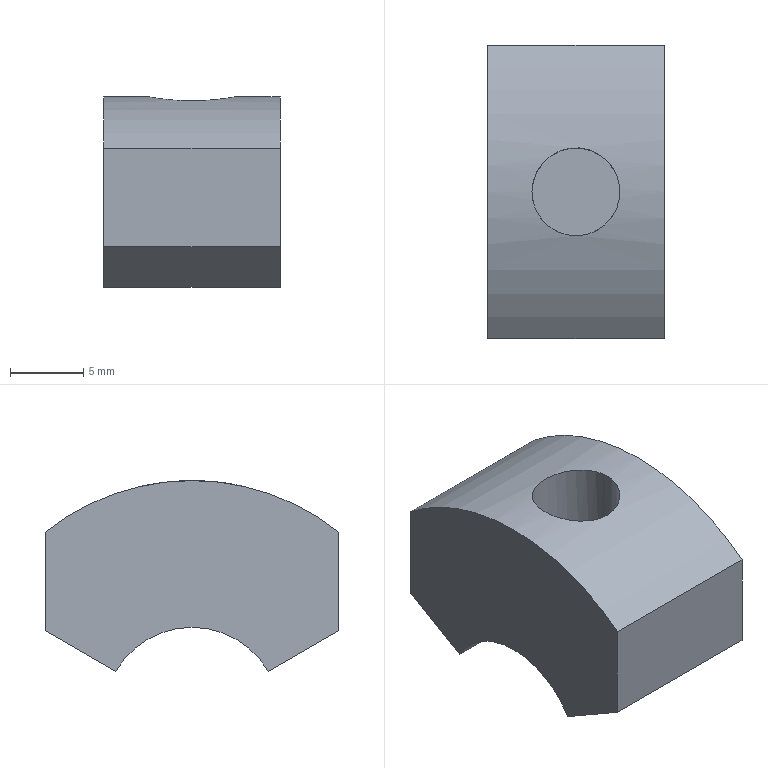Component | NX | BEARING_BUSH | 1 solid | 10 faces | box 12 x 20 x 13 mm | volume 2260 mm3 | plane 7 | cylinder 3 | commonest cylinder face diameters 12 x1 32 x1 6 x1
STEP:
#1=CARTESIAN_POINT('',(0.,0.,0.));
#2=DIRECTION('',(0.,0.,1.));
#3=DIRECTION('',(1.,0.,0.));
#4=AXIS2_PLACEMENT_3D('',#1,#2,#3);
#5=CARTESIAN_POINT('',(6.,10.,48.99));
#6=VERTEX_POINT('',#5);
#7=CARTESIAN_POINT('',(6.,10.,42.274));
#8=VERTEX_POINT('',#7);
#9=CARTESIAN_POINT('',(6.,10.,48.99));
#10=DIRECTION('',(0.,0.,-1.));
#11=VECTOR('',#10,1.);
#12=LINE('',#9,#11);
#13=CARTESIAN_POINT('',(-6.,10.,48.99));
#14=DIRECTION('',(0.,-1.,-0.));
#15=DIRECTION('',(0.,-0.,1.));
#16=AXIS2_PLACEMENT_3D('',#13,#14,#15);
#17=PLANE('',#16);
#18=CARTESIAN_POINT('',(0.,-12.));
#19=DIRECTION('',(-1.,0.));
#20=VECTOR('',#19,1.);
#21=LINE('',#18,#20);
#22=(GEOMETRIC_REPRESENTATION_CONTEXT(2)PARAMETRIC_REPRESENTATION_CONTEXT()REPRESENTATION_CONTEXT('',''));
#23=DEFINITIONAL_REPRESENTATION('',(#21),#22);
#24=PCURVE('',#17,#23);
#25=CARTESIAN_POINT('',(6.,-0.,36.5));
#26=DIRECTION('',(1.,0.,0.));
#27=DIRECTION('',(0.,0.,1.));
#28=AXIS2_PLACEMENT_3D('',#25,#26,#27);
#29=PLANE('',#28);
#30=CARTESIAN_POINT('',(12.49,-10.));
#31=DIRECTION('',(-1.,-0.));
#32=VECTOR('',#31,1.);
#33=LINE('',#30,#32);
#34=(GEOMETRIC_REPRESENTATION_CONTEXT(2)PARAMETRIC_REPRESENTATION_CONTEXT()REPRESENTATION_CONTEXT('',''));
#35=DEFINITIONAL_REPRESENTATION('',(#33),#34);
#36=PCURVE('',#29,#35);
#37=SURFACE_CURVE('',#12,(#24,#36),.PCURVE_S1.);
#38=EDGE_CURVE('',#6,#8,#37,.T.);
#39=ORIENTED_EDGE('',*,*,#38,.T.);
#40=CARTESIAN_POINT('',(-6.,10.,42.274));
#41=VERTEX_POINT('',#40);
#42=CARTESIAN_POINT('',(-6.,10.,42.274));
#43=DIRECTION('',(1.,0.,0.));
#44=VECTOR('',#43,1.);
#45=LINE('',#42,#44);
#46=CARTESIAN_POINT('',(-6.716,0.));
#47=DIRECTION('',(0.,-1.));
#48=VECTOR('',#47,1.);
#49=LINE('',#46,#48);
#50=(GEOMETRIC_REPRESENTATION_CONTEXT(2)PARAMETRIC_REPRESENTATION_CONTEXT()REPRESENTATION_CONTEXT('',''));
#51=DEFINITIONAL_REPRESENTATION('',(#49),#50);
#52=PCURVE('',#17,#51);
#53=CARTESIAN_POINT('',(-6.,10.,42.274));
#54=DIRECTION('',(0.,-0.5,0.866));
#55=DIRECTION('',(0.,0.866,0.5));
#56=AXIS2_PLACEMENT_3D('',#53,#54,#55);
#57=PLANE('',#56);
#58=CARTESIAN_POINT('',(0.,0.));
#59=DIRECTION('',(0.,-1.));
#60=VECTOR('',#59,1.);
#61=LINE('',#58,#60);
#62=(GEOMETRIC_REPRESENTATION_CONTEXT(2)PARAMETRIC_REPRESENTATION_CONTEXT()REPRESENTATION_CONTEXT('',''));
#63=DEFINITIONAL_REPRESENTATION('',(#61),#62);
#64=PCURVE('',#57,#63);
#65=SURFACE_CURVE('',#45,(#52,#64),.PCURVE_S1.);
#66=EDGE_CURVE('',#41,#8,#65,.T.);
#67=ORIENTED_EDGE('',*,*,#66,.F.);
#68=CARTESIAN_POINT('',(-6.,10.,48.99));
#69=VERTEX_POINT('',#68);
#70=CARTESIAN_POINT('',(-6.,10.,48.99));
#71=DIRECTION('',(0.,0.,-1.));
#72=VECTOR('',#71,1.);
#73=LINE('',#70,#72);
#74=CARTESIAN_POINT('',(0.,0.));
#75=DIRECTION('',(-1.,0.));
#76=VECTOR('',#75,1.);
#77=LINE('',#74,#76);
#78=(GEOMETRIC_REPRESENTATION_CONTEXT(2)PARAMETRIC_REPRESENTATION_CONTEXT()REPRESENTATION_CONTEXT('',''));
#79=DEFINITIONAL_REPRESENTATION('',(#77),#78);
#80=PCURVE('',#17,#79);
#81=CARTESIAN_POINT('',(-6.,-0.,36.5));
#82=DIRECTION('',(1.,0.,0.));
#83=DIRECTION('',(0.,0.,1.));
#84=AXIS2_PLACEMENT_3D('',#81,#82,#83);
#85=PLANE('',#84);
#86=CARTESIAN_POINT('',(12.49,-10.));
#87=DIRECTION('',(-1.,-0.));
#88=VECTOR('',#87,1.);
#89=LINE('',#86,#88);
#90=(GEOMETRIC_REPRESENTATION_CONTEXT(2)PARAMETRIC_REPRESENTATION_CONTEXT()REPRESENTATION_CONTEXT('',''));
#91=DEFINITIONAL_REPRESENTATION('',(#89),#90);
#92=PCURVE('',#85,#91);
#93=SURFACE_CURVE('',#73,(#80,#92),.PCURVE_S1.);
#94=EDGE_CURVE('',#69,#41,#93,.T.);
#95=ORIENTED_EDGE('',*,*,#94,.F.);
#96=CARTESIAN_POINT('',(-6.,10.,48.99));
#97=DIRECTION('',(1.,0.,0.));
#98=VECTOR('',#97,1.);
#99=LINE('',#96,#98);
#100=CARTESIAN_POINT('',(0.,0.));
#101=DIRECTION('',(0.,-1.));
#102=VECTOR('',#101,1.);
#103=LINE('',#100,#102);
#104=(GEOMETRIC_REPRESENTATION_CONTEXT(2)PARAMETRIC_REPRESENTATION_CONTEXT()REPRESENTATION_CONTEXT('',''));
#105=DEFINITIONAL_REPRESENTATION('',(#103),#104);
#106=PCURVE('',#17,#105);
#107=CARTESIAN_POINT('',(-6.,-0.,36.5));
#108=DIRECTION('',(1.,0.,0.));
#109=DIRECTION('',(0.,0.,1.));
#110=AXIS2_PLACEMENT_3D('',#107,#108,#109);
#111=CYLINDRICAL_SURFACE('',#110,16.);
#112=CARTESIAN_POINT('',(-0.6751,0.));
#113=DIRECTION('',(0.,1.));
#114=VECTOR('',#113,1.);
#115=LINE('',#112,#114);
#116=(GEOMETRIC_REPRESENTATION_CONTEXT(2)PARAMETRIC_REPRESENTATION_CONTEXT()REPRESENTATION_CONTEXT('',''));
#117=DEFINITIONAL_REPRESENTATION('',(#115),#116);
#118=PCURVE('',#111,#117);
#119=SURFACE_CURVE('',#99,(#106,#118),.PCURVE_S1.);
#120=EDGE_CURVE('',#69,#6,#119,.T.);
#121=ORIENTED_EDGE('',*,*,#120,.T.);
#122=EDGE_LOOP('',(#39,#67,#95,#121));
#123=FACE_BOUND('',#122,.T.);
#124=ADVANCED_FACE('',(#123),#17,.F.);
#125=CARTESIAN_POINT('',(6.,5.196,39.5));
#126=VERTEX_POINT('',#125);
#127=CARTESIAN_POINT('',(6.,10.,42.274));
#128=DIRECTION('',(0.,-0.866,-0.5));
#129=VECTOR('',#128,1.);
#130=LINE('',#127,#129);
#131=CARTESIAN_POINT('',(0.,-12.));
#132=DIRECTION('',(-1.,0.));
#133=VECTOR('',#132,1.);
#134=LINE('',#131,#133);
#135=(GEOMETRIC_REPRESENTATION_CONTEXT(2)PARAMETRIC_REPRESENTATION_CONTEXT()REPRESENTATION_CONTEXT('',''));
#136=DEFINITIONAL_REPRESENTATION('',(#134),#135);
#137=PCURVE('',#57,#136);
#138=CARTESIAN_POINT('',(5.774,-10.));
#139=DIRECTION('',(-0.5,0.866));
#140=VECTOR('',#139,1.);
#141=LINE('',#138,#140);
#142=(GEOMETRIC_REPRESENTATION_CONTEXT(2)PARAMETRIC_REPRESENTATION_CONTEXT()REPRESENTATION_CONTEXT('',''));
#143=DEFINITIONAL_REPRESENTATION('',(#141),#142);
#144=PCURVE('',#29,#143);
#145=SURFACE_CURVE('',#130,(#137,#144),.PCURVE_S1.);
#146=EDGE_CURVE('',#8,#126,#145,.T.);
#147=ORIENTED_EDGE('',*,*,#146,.T.);
#148=CARTESIAN_POINT('',(-6.,5.196,39.5));
#149=VERTEX_POINT('',#148);
#150=CARTESIAN_POINT('',(-6.,5.196,39.5));
#151=DIRECTION('',(1.,0.,0.));
#152=VECTOR('',#151,1.);
#153=LINE('',#150,#152);
#154=CARTESIAN_POINT('',(-5.547,0.));
#155=DIRECTION('',(0.,-1.));
#156=VECTOR('',#155,1.);
#157=LINE('',#154,#156);
#158=(GEOMETRIC_REPRESENTATION_CONTEXT(2)PARAMETRIC_REPRESENTATION_CONTEXT()REPRESENTATION_CONTEXT('',''));
#159=DEFINITIONAL_REPRESENTATION('',(#157),#158);
#160=PCURVE('',#57,#159);
#161=CARTESIAN_POINT('',(-6.,-0.,36.5));
#162=DIRECTION('',(1.,0.,0.));
#163=DIRECTION('',(0.,0.,1.));
#164=AXIS2_PLACEMENT_3D('',#161,#162,#163);
#165=CYLINDRICAL_SURFACE('',#164,6.);
#166=CARTESIAN_POINT('',(5.236,0.));
#167=DIRECTION('',(0.,1.));
#168=VECTOR('',#167,1.);
#169=LINE('',#166,#168);
#170=(GEOMETRIC_REPRESENTATION_CONTEXT(2)PARAMETRIC_REPRESENTATION_CONTEXT()REPRESENTATION_CONTEXT('',''));
#171=DEFINITIONAL_REPRESENTATION('',(#169),#170);
#172=PCURVE('',#165,#171);
#173=SURFACE_CURVE('',#153,(#160,#172),.PCURVE_S1.);
#174=EDGE_CURVE('',#149,#126,#173,.T.);
#175=ORIENTED_EDGE('',*,*,#174,.F.);
#176=CARTESIAN_POINT('',(-6.,10.,42.274));
#177=DIRECTION('',(0.,-0.866,-0.5));
#178=VECTOR('',#177,1.);
#179=LINE('',#176,#178);
#180=CARTESIAN_POINT('',(0.,0.));
#181=DIRECTION('',(-1.,0.));
#182=VECTOR('',#181,1.);
#183=LINE('',#180,#182);
#184=(GEOMETRIC_REPRESENTATION_CONTEXT(2)PARAMETRIC_REPRESENTATION_CONTEXT()REPRESENTATION_CONTEXT('',''));
#185=DEFINITIONAL_REPRESENTATION('',(#183),#184);
#186=PCURVE('',#57,#185);
#187=CARTESIAN_POINT('',(5.774,-10.));
#188=DIRECTION('',(-0.5,0.866));
#189=VECTOR('',#188,1.);
#190=LINE('',#187,#189);
#191=(GEOMETRIC_REPRESENTATION_CONTEXT(2)PARAMETRIC_REPRESENTATION_CONTEXT()REPRESENTATION_CONTEXT('',''));
#192=DEFINITIONAL_REPRESENTATION('',(#190),#191);
#193=PCURVE('',#85,#192);
#194=SURFACE_CURVE('',#179,(#186,#193),.PCURVE_S1.);
#195=EDGE_CURVE('',#41,#149,#194,.T.);
#196=ORIENTED_EDGE('',*,*,#195,.F.);
#197=ORIENTED_EDGE('',*,*,#66,.T.);
#198=EDGE_LOOP('',(#147,#175,#196,#197));
#199=FACE_BOUND('',#198,.T.);
#200=ADVANCED_FACE('',(#199),#57,.F.);
#201=ORIENTED_EDGE('',*,*,#174,.F.);
#202=CARTESIAN_POINT('',(-6.,-5.196,39.5));
#203=VERTEX_POINT('',#202);
#204=CARTESIAN_POINT('',(-6.,-0.,36.5));
#205=DIRECTION('',(1.,0.,0.));
#206=DIRECTION('',(0.,-1.,0.));
#207=AXIS2_PLACEMENT_3D('',#204,#205,#206);
#208=CIRCLE('',#207,6.);
#209=CARTESIAN_POINT('',(1.571,0.));
#210=DIRECTION('',(1.,0.));
#211=VECTOR('',#210,1.);
#212=LINE('',#209,#211);
#213=(GEOMETRIC_REPRESENTATION_CONTEXT(2)PARAMETRIC_REPRESENTATION_CONTEXT()REPRESENTATION_CONTEXT('',''));
#214=DEFINITIONAL_REPRESENTATION('',(#212),#213);
#215=PCURVE('',#165,#214);
#216=CARTESIAN_POINT('',(0.,0.));
#217=DIRECTION('',(0.,1.));
#218=AXIS2_PLACEMENT_2D('',#216,#217);
#219=CIRCLE('',#218,6.);
#220=(GEOMETRIC_REPRESENTATION_CONTEXT(2)PARAMETRIC_REPRESENTATION_CONTEXT()REPRESENTATION_CONTEXT('',''));
#221=DEFINITIONAL_REPRESENTATION('',(#219),#220);
#222=PCURVE('',#85,#221);
#223=SURFACE_CURVE('',#208,(#215,#222),.PCURVE_S1.);
#224=EDGE_CURVE('',#149,#203,#223,.T.);
#225=ORIENTED_EDGE('',*,*,#224,.T.);
#226=CARTESIAN_POINT('',(6.,-5.196,39.5));
#227=VERTEX_POINT('',#226);
#228=CARTESIAN_POINT('',(-6.,-5.196,39.5));
#229=DIRECTION('',(1.,0.,0.));
#230=VECTOR('',#229,1.);
#231=LINE('',#228,#230);
#232=CARTESIAN_POINT('',(7.33,0.));
#233=DIRECTION('',(0.,1.));
#234=VECTOR('',#233,1.);
#235=LINE('',#232,#234);
#236=(GEOMETRIC_REPRESENTATION_CONTEXT(2)PARAMETRIC_REPRESENTATION_CONTEXT()REPRESENTATION_CONTEXT('',''));
#237=DEFINITIONAL_REPRESENTATION('',(#235),#236);
#238=PCURVE('',#165,#237);
#239=CARTESIAN_POINT('',(-6.,-5.196,39.5));
#240=DIRECTION('',(0.,0.5,0.866));
#241=DIRECTION('',(0.,0.866,-0.5));
#242=AXIS2_PLACEMENT_3D('',#239,#240,#241);
#243=PLANE('',#242);
#244=CARTESIAN_POINT('',(0.,0.));
#245=DIRECTION('',(0.,-1.));
#246=VECTOR('',#245,1.);
#247=LINE('',#244,#246);
#248=(GEOMETRIC_REPRESENTATION_CONTEXT(2)PARAMETRIC_REPRESENTATION_CONTEXT()REPRESENTATION_CONTEXT('',''));
#249=DEFINITIONAL_REPRESENTATION('',(#247),#248);
#250=PCURVE('',#243,#249);
#251=SURFACE_CURVE('',#231,(#238,#250),.PCURVE_S1.);
#252=EDGE_CURVE('',#203,#227,#251,.T.);
#253=ORIENTED_EDGE('',*,*,#252,.T.);
#254=CARTESIAN_POINT('',(6.,-0.,36.5));
#255=DIRECTION('',(1.,0.,0.));
#256=DIRECTION('',(0.,-1.,0.));
#257=AXIS2_PLACEMENT_3D('',#254,#255,#256);
#258=CIRCLE('',#257,6.);
#259=CARTESIAN_POINT('',(1.571,12.));
#260=DIRECTION('',(1.,0.));
#261=VECTOR('',#260,1.);
#262=LINE('',#259,#261);
#263=(GEOMETRIC_REPRESENTATION_CONTEXT(2)PARAMETRIC_REPRESENTATION_CONTEXT()REPRESENTATION_CONTEXT('',''));
#264=DEFINITIONAL_REPRESENTATION('',(#262),#263);
#265=PCURVE('',#165,#264);
#266=CARTESIAN_POINT('',(0.,0.));
#267=DIRECTION('',(0.,1.));
#268=AXIS2_PLACEMENT_2D('',#266,#267);
#269=CIRCLE('',#268,6.);
#270=(GEOMETRIC_REPRESENTATION_CONTEXT(2)PARAMETRIC_REPRESENTATION_CONTEXT()REPRESENTATION_CONTEXT('',''));
#271=DEFINITIONAL_REPRESENTATION('',(#269),#270);
#272=PCURVE('',#29,#271);
#273=SURFACE_CURVE('',#258,(#265,#272),.PCURVE_S1.);
#274=EDGE_CURVE('',#126,#227,#273,.T.);
#275=ORIENTED_EDGE('',*,*,#274,.F.);
#276=EDGE_LOOP('',(#201,#225,#253,#275));
#277=FACE_BOUND('',#276,.F.);
#278=ADVANCED_FACE('',(#277),#165,.F.);
#279=CARTESIAN_POINT('',(6.,-10.,42.274));
#280=VERTEX_POINT('',#279);
#281=CARTESIAN_POINT('',(6.,-5.196,39.5));
#282=DIRECTION('',(0.,-0.866,0.5));
#283=VECTOR('',#282,1.);
#284=LINE('',#281,#283);
#285=CARTESIAN_POINT('',(0.,-12.));
#286=DIRECTION('',(-1.,0.));
#287=VECTOR('',#286,1.);
#288=LINE('',#285,#287);
#289=(GEOMETRIC_REPRESENTATION_CONTEXT(2)PARAMETRIC_REPRESENTATION_CONTEXT()REPRESENTATION_CONTEXT('',''));
#290=DEFINITIONAL_REPRESENTATION('',(#288),#289);
#291=PCURVE('',#243,#290);
#292=CARTESIAN_POINT('',(3.,5.196));
#293=DIRECTION('',(0.5,0.866));
#294=VECTOR('',#293,1.);
#295=LINE('',#292,#294);
#296=(GEOMETRIC_REPRESENTATION_CONTEXT(2)PARAMETRIC_REPRESENTATION_CONTEXT()REPRESENTATION_CONTEXT('',''));
#297=DEFINITIONAL_REPRESENTATION('',(#295),#296);
#298=PCURVE('',#29,#297);
#299=SURFACE_CURVE('',#284,(#291,#298),.PCURVE_S1.);
#300=EDGE_CURVE('',#227,#280,#299,.T.);
#301=ORIENTED_EDGE('',*,*,#300,.T.);
#302=CARTESIAN_POINT('',(-6.,-10.,42.274));
#303=VERTEX_POINT('',#302);
#304=CARTESIAN_POINT('',(-6.,-10.,42.274));
#305=DIRECTION('',(1.,0.,0.));
#306=VECTOR('',#305,1.);
#307=LINE('',#304,#306);
#308=CARTESIAN_POINT('',(-5.547,0.));
#309=DIRECTION('',(0.,-1.));
#310=VECTOR('',#309,1.);
#311=LINE('',#308,#310);
#312=(GEOMETRIC_REPRESENTATION_CONTEXT(2)PARAMETRIC_REPRESENTATION_CONTEXT()REPRESENTATION_CONTEXT('',''));
#313=DEFINITIONAL_REPRESENTATION('',(#311),#312);
#314=PCURVE('',#243,#313);
#315=CARTESIAN_POINT('',(-6.,-10.,42.274));
#316=DIRECTION('',(0.,1.,-0.));
#317=DIRECTION('',(0.,-0.,-1.));
#318=AXIS2_PLACEMENT_3D('',#315,#316,#317);
#319=PLANE('',#318);
#320=CARTESIAN_POINT('',(0.,0.));
#321=DIRECTION('',(0.,-1.));
#322=VECTOR('',#321,1.);
#323=LINE('',#320,#322);
#324=(GEOMETRIC_REPRESENTATION_CONTEXT(2)PARAMETRIC_REPRESENTATION_CONTEXT()REPRESENTATION_CONTEXT('',''));
#325=DEFINITIONAL_REPRESENTATION('',(#323),#324);
#326=PCURVE('',#319,#325);
#327=SURFACE_CURVE('',#307,(#314,#326),.PCURVE_S1.);
#328=EDGE_CURVE('',#303,#280,#327,.T.);
#329=ORIENTED_EDGE('',*,*,#328,.F.);
#330=CARTESIAN_POINT('',(-6.,-5.196,39.5));
#331=DIRECTION('',(0.,-0.866,0.5));
#332=VECTOR('',#331,1.);
#333=LINE('',#330,#332);
#334=CARTESIAN_POINT('',(0.,0.));
#335=DIRECTION('',(-1.,0.));
#336=VECTOR('',#335,1.);
#337=LINE('',#334,#336);
#338=(GEOMETRIC_REPRESENTATION_CONTEXT(2)PARAMETRIC_REPRESENTATION_CONTEXT()REPRESENTATION_CONTEXT('',''));
#339=DEFINITIONAL_REPRESENTATION('',(#337),#338);
#340=PCURVE('',#243,#339);
#341=CARTESIAN_POINT('',(3.,5.196));
#342=DIRECTION('',(0.5,0.866));
#343=VECTOR('',#342,1.);
#344=LINE('',#341,#343);
#345=(GEOMETRIC_REPRESENTATION_CONTEXT(2)PARAMETRIC_REPRESENTATION_CONTEXT()REPRESENTATION_CONTEXT('',''));
#346=DEFINITIONAL_REPRESENTATION('',(#344),#345);
#347=PCURVE('',#85,#346);
#348=SURFACE_CURVE('',#333,(#340,#347),.PCURVE_S1.);
#349=EDGE_CURVE('',#203,#303,#348,.T.);
#350=ORIENTED_EDGE('',*,*,#349,.F.);
#351=ORIENTED_EDGE('',*,*,#252,.T.);
#352=EDGE_LOOP('',(#301,#329,#350,#351));
#353=FACE_BOUND('',#352,.T.);
#354=ADVANCED_FACE('',(#353),#243,.F.);
#355=CARTESIAN_POINT('',(6.,-10.,48.99));
#356=VERTEX_POINT('',#355);
#357=CARTESIAN_POINT('',(6.,-10.,42.274));
#358=DIRECTION('',(0.,0.,1.));
#359=VECTOR('',#358,1.);
#360=LINE('',#357,#359);
#361=CARTESIAN_POINT('',(0.,-12.));
#362=DIRECTION('',(-1.,0.));
#363=VECTOR('',#362,1.);
#364=LINE('',#361,#363);
#365=(GEOMETRIC_REPRESENTATION_CONTEXT(2)PARAMETRIC_REPRESENTATION_CONTEXT()REPRESENTATION_CONTEXT('',''));
#366=DEFINITIONAL_REPRESENTATION('',(#364),#365);
#367=PCURVE('',#319,#366);
#368=CARTESIAN_POINT('',(5.774,10.));
#369=DIRECTION('',(1.,-0.));
#370=VECTOR('',#369,1.);
#371=LINE('',#368,#370);
#372=(GEOMETRIC_REPRESENTATION_CONTEXT(2)PARAMETRIC_REPRESENTATION_CONTEXT()REPRESENTATION_CONTEXT('',''));
#373=DEFINITIONAL_REPRESENTATION('',(#371),#372);
#374=PCURVE('',#29,#373);
#375=SURFACE_CURVE('',#360,(#367,#374),.PCURVE_S1.);
#376=EDGE_CURVE('',#280,#356,#375,.T.);
#377=ORIENTED_EDGE('',*,*,#376,.T.);
#378=CARTESIAN_POINT('',(-6.,-10.,48.99));
#379=VERTEX_POINT('',#378);
#380=CARTESIAN_POINT('',(-6.,-10.,48.99));
#381=DIRECTION('',(1.,0.,0.));
#382=VECTOR('',#381,1.);
#383=LINE('',#380,#382);
#384=CARTESIAN_POINT('',(-6.716,0.));
#385=DIRECTION('',(0.,-1.));
#386=VECTOR('',#385,1.);
#387=LINE('',#384,#386);
#388=(GEOMETRIC_REPRESENTATION_CONTEXT(2)PARAMETRIC_REPRESENTATION_CONTEXT()REPRESENTATION_CONTEXT('',''));
#389=DEFINITIONAL_REPRESENTATION('',(#387),#388);
#390=PCURVE('',#319,#389);
#391=CARTESIAN_POINT('',(0.6751,0.));
#392=DIRECTION('',(0.,1.));
#393=VECTOR('',#392,1.);
#394=LINE('',#391,#393);
#395=(GEOMETRIC_REPRESENTATION_CONTEXT(2)PARAMETRIC_REPRESENTATION_CONTEXT()REPRESENTATION_CONTEXT('',''));
#396=DEFINITIONAL_REPRESENTATION('',(#394),#395);
#397=PCURVE('',#111,#396);
#398=SURFACE_CURVE('',#383,(#390,#397),.PCURVE_S1.);
#399=EDGE_CURVE('',#379,#356,#398,.T.);
#400=ORIENTED_EDGE('',*,*,#399,.F.);
#401=CARTESIAN_POINT('',(-6.,-10.,42.274));
#402=DIRECTION('',(0.,0.,1.));
#403=VECTOR('',#402,1.);
#404=LINE('',#401,#403);
#405=CARTESIAN_POINT('',(0.,0.));
#406=DIRECTION('',(-1.,0.));
#407=VECTOR('',#406,1.);
#408=LINE('',#405,#407);
#409=(GEOMETRIC_REPRESENTATION_CONTEXT(2)PARAMETRIC_REPRESENTATION_CONTEXT()REPRESENTATION_CONTEXT('',''));
#410=DEFINITIONAL_REPRESENTATION('',(#408),#409);
#411=PCURVE('',#319,#410);
#412=CARTESIAN_POINT('',(5.774,10.));
#413=DIRECTION('',(1.,-0.));
#414=VECTOR('',#413,1.);
#415=LINE('',#412,#414);
#416=(GEOMETRIC_REPRESENTATION_CONTEXT(2)PARAMETRIC_REPRESENTATION_CONTEXT()REPRESENTATION_CONTEXT('',''));
#417=DEFINITIONAL_REPRESENTATION('',(#415),#416);
#418=PCURVE('',#85,#417);
#419=SURFACE_CURVE('',#404,(#411,#418),.PCURVE_S1.);
#420=EDGE_CURVE('',#303,#379,#419,.T.);
#421=ORIENTED_EDGE('',*,*,#420,.F.);
#422=ORIENTED_EDGE('',*,*,#328,.T.);
#423=EDGE_LOOP('',(#377,#400,#421,#422));
#424=FACE_BOUND('',#423,.T.);
#425=ADVANCED_FACE('',(#424),#319,.F.);
#426=CARTESIAN_POINT('',(-3.,-0.,52.5));
#427=VERTEX_POINT('',#426);
#428=CARTESIAN_POINT('',(-3.,-0.,52.5));
#429=CARTESIAN_POINT('',(-3.,0.3325,52.5));
#430=CARTESIAN_POINT('',(-2.943,0.6696,52.489));
#431=CARTESIAN_POINT('',(-2.834,0.9833,52.47));
#432=CARTESIAN_POINT('',(-2.726,1.297,52.45));
#433=CARTESIAN_POINT('',(-2.562,1.595,52.422));
#434=CARTESIAN_POINT('',(-2.357,1.856,52.392));
#435=CARTESIAN_POINT('',(-2.15,2.118,52.361));
#436=CARTESIAN_POINT('',(-1.896,2.349,52.328));
#437=CARTESIAN_POINT('',(-1.614,2.529,52.299));
#438=CARTESIAN_POINT('',(-1.329,2.711,52.27));
#439=CARTESIAN_POINT('',(-1.009,2.845,52.245));
#440=CARTESIAN_POINT('',(-0.6794,2.922,52.231));
#441=CARTESIAN_POINT('',(-0.3538,2.998,52.217));
#442=CARTESIAN_POINT('',(-0.01006,3.019,52.213));
#443=CARTESIAN_POINT('',(0.3225,2.983,52.22));
#444=CARTESIAN_POINT('',(0.6508,2.947,52.226));
#445=CARTESIAN_POINT('',(0.9772,2.855,52.244));
#446=CARTESIAN_POINT('',(1.275,2.715,52.268));
#447=CARTESIAN_POINT('',(1.575,2.575,52.292));
#448=CARTESIAN_POINT('',(1.855,2.381,52.324));
#449=CARTESIAN_POINT('',(2.092,2.15,52.355));
#450=CARTESIAN_POINT('',(2.333,1.916,52.387));
#451=CARTESIAN_POINT('',(2.536,1.637,52.419));
#452=CARTESIAN_POINT('',(2.686,1.336,52.444));
#453=CARTESIAN_POINT('',(2.836,1.034,52.469));
#454=CARTESIAN_POINT('',(2.936,0.7015,52.488));
#455=CARTESIAN_POINT('',(2.978,0.3662,52.496));
#456=CARTESIAN_POINT('',(3.018,0.03596,52.503));
#457=CARTESIAN_POINT('',(3.003,-0.3061,52.5));
#458=CARTESIAN_POINT('',(2.933,-0.6313,52.488));
#459=CARTESIAN_POINT('',(2.863,-0.9539,52.475));
#460=CARTESIAN_POINT('',(2.738,-1.269,52.452));
#461=CARTESIAN_POINT('',(2.568,-1.551,52.425));
#462=CARTESIAN_POINT('',(2.396,-1.835,52.397));
#463=CARTESIAN_POINT('',(2.173,-2.094,52.364));
#464=CARTESIAN_POINT('',(1.918,-2.307,52.333));
#465=CARTESIAN_POINT('',(1.659,-2.522,52.301));
#466=CARTESIAN_POINT('',(1.359,-2.696,52.272));
#467=CARTESIAN_POINT('',(1.042,-2.813,52.251));
#468=CARTESIAN_POINT('',(0.7268,-2.93,52.23));
#469=CARTESIAN_POINT('',(0.3865,-2.994,52.217));
#470=CARTESIAN_POINT('',(0.04993,-3.,52.216));
#471=CARTESIAN_POINT('',(-0.2813,-3.005,52.215));
#472=CARTESIAN_POINT('',(-0.6181,-2.954,52.225));
#473=CARTESIAN_POINT('',(-0.9325,-2.851,52.244));
#474=CARTESIAN_POINT('',(-1.246,-2.749,52.262));
#475=CARTESIAN_POINT('',(-1.546,-2.592,52.29));
#476=CARTESIAN_POINT('',(-1.809,-2.393,52.32));
#477=CARTESIAN_POINT('',(-2.076,-2.191,52.351));
#478=CARTESIAN_POINT('',(-2.311,-1.941,52.384));
#479=CARTESIAN_POINT('',(-2.497,-1.663,52.413));
#480=CARTESIAN_POINT('',(-2.684,-1.382,52.443));
#481=CARTESIAN_POINT('',(-2.825,-1.065,52.468));
#482=CARTESIAN_POINT('',(-2.908,-0.7369,52.483));
#483=CARTESIAN_POINT('',(-2.969,-0.4971,52.494));
#484=CARTESIAN_POINT('',(-3.,-0.2476,52.5));
#485=CARTESIAN_POINT('',(-3.,-0.,52.5));
#486=B_SPLINE_CURVE_WITH_KNOTS('',3,(#428,#429,#430,#431,#432,#433,#434,#435,#436,#437,#438,#439,#440,#441,#442,#443,#444,#445,#446,#447,#448,#449,#450,#451,#452,#453,#454,#455,#456,#457,#458,#459,#460,#461,#462,#463,#464,#465,#466,#467,#468,#469,#470,#471,#472,#473,#474,#475,#476,#477,#478,#479,#480,#481,#482,#483,#484,#485),.UNSPECIFIED.,.T.,.F.,(1,3,3,3,3,3,3,3,3,3,3,3,3,3,3,3,3,3,3,3,3,1),(-0.03926,0.,0.05307,0.1061,0.1597,0.2138,0.2672,0.3199,0.3729,0.4267,0.4807,0.5338,0.5865,0.6397,0.6938,0.7475,0.8004,0.8531,0.9067,0.9607,1.,1.053),.UNSPECIFIED.);
#487=CARTESIAN_POINT('',(0.,3.));
#488=CARTESIAN_POINT('',(-0.00445,3.));
#489=CARTESIAN_POINT('',(-0.01338,3.005));
#490=CARTESIAN_POINT('',(-0.02675,3.028));
#491=CARTESIAN_POINT('',(-0.03999,3.067));
#492=CARTESIAN_POINT('',(-0.05301,3.12));
#493=CARTESIAN_POINT('',(-0.06569,3.187));
#494=CARTESIAN_POINT('',(-0.07809,3.269));
#495=CARTESIAN_POINT('',(-0.09012,3.366));
#496=CARTESIAN_POINT('',(-0.1017,3.475));
#497=CARTESIAN_POINT('',(-0.1128,3.597));
#498=CARTESIAN_POINT('',(-0.1232,3.731));
#499=CARTESIAN_POINT('',(-0.133,3.877));
#500=CARTESIAN_POINT('',(-0.1423,4.034));
#501=CARTESIAN_POINT('',(-0.1508,4.2));
#502=CARTESIAN_POINT('',(-0.1585,4.375));
#503=CARTESIAN_POINT('',(-0.1654,4.559));
#504=CARTESIAN_POINT('',(-0.1715,4.751));
#505=CARTESIAN_POINT('',(-0.1767,4.949));
#506=CARTESIAN_POINT('',(-0.181,5.153));
#507=CARTESIAN_POINT('',(-0.1844,5.359));
#508=CARTESIAN_POINT('',(-0.1868,5.57));
#509=CARTESIAN_POINT('',(-0.1883,5.784));
#510=CARTESIAN_POINT('',(-0.1888,5.999));
#511=CARTESIAN_POINT('',(-0.1883,6.214));
#512=CARTESIAN_POINT('',(-0.1868,6.427));
#513=CARTESIAN_POINT('',(-0.1844,6.638));
#514=CARTESIAN_POINT('',(-0.181,6.846));
#515=CARTESIAN_POINT('',(-0.1767,7.05));
#516=CARTESIAN_POINT('',(-0.1715,7.248));
#517=CARTESIAN_POINT('',(-0.1655,7.439));
#518=CARTESIAN_POINT('',(-0.1585,7.623));
#519=CARTESIAN_POINT('',(-0.1508,7.799));
#520=CARTESIAN_POINT('',(-0.1423,7.966));
#521=CARTESIAN_POINT('',(-0.1331,8.122));
#522=CARTESIAN_POINT('',(-0.1233,8.268));
#523=CARTESIAN_POINT('',(-0.1128,8.402));
#524=CARTESIAN_POINT('',(-0.1017,8.525));
#525=CARTESIAN_POINT('',(-0.09018,8.634));
#526=CARTESIAN_POINT('',(-0.07824,8.73));
#527=CARTESIAN_POINT('',(-0.06583,8.812));
#528=CARTESIAN_POINT('',(-0.05307,8.88));
#529=CARTESIAN_POINT('',(-0.04004,8.933));
#530=CARTESIAN_POINT('',(-0.02685,8.972));
#531=CARTESIAN_POINT('',(-0.01357,8.995));
#532=CARTESIAN_POINT('',(-0.0001349,9.002));
#533=CARTESIAN_POINT('',(0.01331,8.995));
#534=CARTESIAN_POINT('',(0.02669,8.972));
#535=CARTESIAN_POINT('',(0.03986,8.934));
#536=CARTESIAN_POINT('',(0.05283,8.881));
#537=CARTESIAN_POINT('',(0.0656,8.813));
#538=CARTESIAN_POINT('',(0.07804,8.731));
#539=CARTESIAN_POINT('',(0.09007,8.635));
#540=CARTESIAN_POINT('',(0.1016,8.526));
#541=CARTESIAN_POINT('',(0.1126,8.404));
#542=CARTESIAN_POINT('',(0.1231,8.27));
#543=CARTESIAN_POINT('',(0.133,8.124));
#544=CARTESIAN_POINT('',(0.1422,7.968));
#545=CARTESIAN_POINT('',(0.1507,7.802));
#546=CARTESIAN_POINT('',(0.1584,7.626));
#547=CARTESIAN_POINT('',(0.1653,7.442));
#548=CARTESIAN_POINT('',(0.1714,7.25));
#549=CARTESIAN_POINT('',(0.1767,7.053));
#550=CARTESIAN_POINT('',(0.181,6.85));
#551=CARTESIAN_POINT('',(0.1843,6.642));
#552=CARTESIAN_POINT('',(0.1868,6.43));
#553=CARTESIAN_POINT('',(0.1883,6.217));
#554=CARTESIAN_POINT('',(0.1888,6.003));
#555=CARTESIAN_POINT('',(0.1883,5.789));
#556=CARTESIAN_POINT('',(0.1868,5.575));
#557=CARTESIAN_POINT('',(0.1844,5.363));
#558=CARTESIAN_POINT('',(0.1811,5.155));
#559=CARTESIAN_POINT('',(0.1768,4.952));
#560=CARTESIAN_POINT('',(0.1716,4.754));
#561=CARTESIAN_POINT('',(0.1655,4.562));
#562=CARTESIAN_POINT('',(0.1585,4.377));
#563=CARTESIAN_POINT('',(0.1509,4.202));
#564=CARTESIAN_POINT('',(0.1424,4.036));
#565=CARTESIAN_POINT('',(0.1332,3.879));
#566=CARTESIAN_POINT('',(0.1233,3.733));
#567=CARTESIAN_POINT('',(0.1128,3.598));
#568=CARTESIAN_POINT('',(0.1019,3.476));
#569=CARTESIAN_POINT('',(0.09032,3.367));
#570=CARTESIAN_POINT('',(0.07829,3.271));
#571=CARTESIAN_POINT('',(0.06586,3.188));
#572=CARTESIAN_POINT('',(0.05314,3.12));
#573=CARTESIAN_POINT('',(0.04017,3.067));
#574=CARTESIAN_POINT('',(0.02688,3.028));
#575=CARTESIAN_POINT('',(0.01346,3.005));
#576=CARTESIAN_POINT('',(0.004479,3.));
#577=CARTESIAN_POINT('',(0.,3.));
#578=B_SPLINE_CURVE_WITH_KNOTS('',3,(#487,#488,#489,#490,#491,#492,#493,#494,#495,#496,#497,#498,#499,#500,#501,#502,#503,#504,#505,#506,#507,#508,#509,#510,#511,#512,#513,#514,#515,#516,#517,#518,#519,#520,#521,#522,#523,#524,#525,#526,#527,#528,#529,#530,#531,#532,#533,#534,#535,#536,#537,#538,#539,#540,#541,#542,#543,#544,#545,#546,#547,#548,#549,#550,#551,#552,#553,#554,#555,#556,#557,#558,#559,#560,#561,#562,#563,#564,#565,#566,#567,#568,#569,#570,#571,#572,#573,#574,#575,#576,#577),.UNSPECIFIED.,.T.,.F.,(4,1,1,1,1,1,1,1,1,1,1,1,1,1,1,1,1,1,1,1,1,1,1,1,1,1,1,1,1,1,1,1,1,1,1,1,1,1,1,1,1,1,1,1,1,1,1,1,1,1,1,1,1,1,1,1,1,1,1,1,1,1,1,1,1,1,1,1,1,1,1,1,1,1,1,1,1,1,1,1,1,1,1,1,1,1,1,1,4),(0.,0.01136,0.02273,0.03409,0.04545,0.05682,0.06818,0.07955,0.09091,0.1023,0.1136,0.125,0.1364,0.1477,0.1591,0.1705,0.1818,0.1932,0.2045,0.2159,0.2273,0.2386,0.25,0.2614,0.2727,0.2841,0.2955,0.3068,0.3182,0.3295,0.3409,0.3523,0.3636,0.375,0.3864,0.3977,0.4091,0.4205,0.4318,0.4432,0.4545,0.4659,0.4773,0.4886,0.5,0.5114,0.5227,0.5341,0.5455,0.5568,0.5682,0.5795,0.5909,0.6023,0.6136,0.625,0.6364,0.6477,0.6591,0.6705,0.6818,0.6932,0.7045,0.7159,0.7273,0.7386,0.75,0.7614,0.7727,0.7841,0.7955,0.8068,0.8182,0.8295,0.8409,0.8523,0.8636,0.875,0.8864,0.8977,0.9091,0.9205,0.9318,0.9432,0.9545,0.9659,0.9773,0.9886,1.),.QUASI_UNIFORM_KNOTS.);
#579=(GEOMETRIC_REPRESENTATION_CONTEXT(2)PARAMETRIC_REPRESENTATION_CONTEXT()REPRESENTATION_CONTEXT('',''));
#580=DEFINITIONAL_REPRESENTATION('',(#578),#579);
#581=PCURVE('',#111,#580);
#582=CARTESIAN_POINT('',(0.,-0.,46.5));
#583=DIRECTION('',(0.,0.,1.));
#584=DIRECTION('',(-1.,0.,0.));
#585=AXIS2_PLACEMENT_3D('',#582,#583,#584);
#586=CYLINDRICAL_SURFACE('',#585,3.);
#587=CARTESIAN_POINT('',(6.283,6.));
#588=CARTESIAN_POINT('',(6.259,6.));
#589=CARTESIAN_POINT('',(6.212,5.999));
#590=CARTESIAN_POINT('',(6.14,5.995));
#591=CARTESIAN_POINT('',(6.068,5.988));
#592=CARTESIAN_POINT('',(5.997,5.978));
#593=CARTESIAN_POINT('',(5.926,5.966));
#594=CARTESIAN_POINT('',(5.854,5.952));
#595=CARTESIAN_POINT('',(5.783,5.935));
#596=CARTESIAN_POINT('',(5.711,5.918));
#597=CARTESIAN_POINT('',(5.64,5.899));
#598=CARTESIAN_POINT('',(5.569,5.879));
#599=CARTESIAN_POINT('',(5.498,5.859));
#600=CARTESIAN_POINT('',(5.427,5.839));
#601=CARTESIAN_POINT('',(5.355,5.819));
#602=CARTESIAN_POINT('',(5.284,5.8));
#603=CARTESIAN_POINT('',(5.213,5.782));
#604=CARTESIAN_POINT('',(5.142,5.766));
#605=CARTESIAN_POINT('',(5.07,5.751));
#606=CARTESIAN_POINT('',(4.998,5.739));
#607=CARTESIAN_POINT('',(4.927,5.729));
#608=CARTESIAN_POINT('',(4.856,5.722));
#609=CARTESIAN_POINT('',(4.784,5.717));
#610=CARTESIAN_POINT('',(4.713,5.716));
#611=CARTESIAN_POINT('',(4.641,5.717));
#612=CARTESIAN_POINT('',(4.57,5.722));
#613=CARTESIAN_POINT('',(4.498,5.729));
#614=CARTESIAN_POINT('',(4.427,5.739));
#615=CARTESIAN_POINT('',(4.355,5.751));
#616=CARTESIAN_POINT('',(4.284,5.765));
#617=CARTESIAN_POINT('',(4.213,5.782));
#618=CARTESIAN_POINT('',(4.141,5.8));
#619=CARTESIAN_POINT('',(4.07,5.819));
#620=CARTESIAN_POINT('',(3.998,5.838));
#621=CARTESIAN_POINT('',(3.927,5.859));
#622=CARTESIAN_POINT('',(3.856,5.879));
#623=CARTESIAN_POINT('',(3.785,5.899));
#624=CARTESIAN_POINT('',(3.713,5.918));
#625=CARTESIAN_POINT('',(3.642,5.935));
#626=CARTESIAN_POINT('',(3.571,5.951));
#627=CARTESIAN_POINT('',(3.5,5.966));
#628=CARTESIAN_POINT('',(3.428,5.978));
#629=CARTESIAN_POINT('',(3.357,5.988));
#630=CARTESIAN_POINT('',(3.285,5.995));
#631=CARTESIAN_POINT('',(3.214,5.999));
#632=CARTESIAN_POINT('',(3.142,6.));
#633=CARTESIAN_POINT('',(3.071,5.999));
#634=CARTESIAN_POINT('',(2.999,5.995));
#635=CARTESIAN_POINT('',(2.928,5.988));
#636=CARTESIAN_POINT('',(2.856,5.978));
#637=CARTESIAN_POINT('',(2.785,5.966));
#638=CARTESIAN_POINT('',(2.713,5.952));
#639=CARTESIAN_POINT('',(2.642,5.936));
#640=CARTESIAN_POINT('',(2.571,5.918));
#641=CARTESIAN_POINT('',(2.499,5.899));
#642=CARTESIAN_POINT('',(2.428,5.879));
#643=CARTESIAN_POINT('',(2.357,5.859));
#644=CARTESIAN_POINT('',(2.285,5.839));
#645=CARTESIAN_POINT('',(2.215,5.819));
#646=CARTESIAN_POINT('',(2.143,5.8));
#647=CARTESIAN_POINT('',(2.072,5.782));
#648=CARTESIAN_POINT('',(2.,5.766));
#649=CARTESIAN_POINT('',(1.929,5.751));
#650=CARTESIAN_POINT('',(1.858,5.739));
#651=CARTESIAN_POINT('',(1.786,5.729));
#652=CARTESIAN_POINT('',(1.715,5.722));
#653=CARTESIAN_POINT('',(1.643,5.717));
#654=CARTESIAN_POINT('',(1.572,5.716));
#655=CARTESIAN_POINT('',(1.5,5.717));
#656=CARTESIAN_POINT('',(1.429,5.722));
#657=CARTESIAN_POINT('',(1.357,5.729));
#658=CARTESIAN_POINT('',(1.285,5.738));
#659=CARTESIAN_POINT('',(1.214,5.751));
#660=CARTESIAN_POINT('',(1.143,5.765));
#661=CARTESIAN_POINT('',(1.071,5.782));
#662=CARTESIAN_POINT('',(0.9999,5.799));
#663=CARTESIAN_POINT('',(0.9287,5.818));
#664=CARTESIAN_POINT('',(0.8577,5.838));
#665=CARTESIAN_POINT('',(0.7864,5.858));
#666=CARTESIAN_POINT('',(0.715,5.879));
#667=CARTESIAN_POINT('',(0.6436,5.899));
#668=CARTESIAN_POINT('',(0.5726,5.917));
#669=CARTESIAN_POINT('',(0.5015,5.935));
#670=CARTESIAN_POINT('',(0.43,5.951));
#671=CARTESIAN_POINT('',(0.3584,5.966));
#672=CARTESIAN_POINT('',(0.287,5.978));
#673=CARTESIAN_POINT('',(0.2157,5.988));
#674=CARTESIAN_POINT('',(0.1437,5.995));
#675=CARTESIAN_POINT('',(0.07178,5.999));
#676=CARTESIAN_POINT('',(0.02389,6.));
#677=CARTESIAN_POINT('',(0.,6.));
#678=B_SPLINE_CURVE_WITH_KNOTS('',3,(#587,#588,#589,#590,#591,#592,#593,#594,#595,#596,#597,#598,#599,#600,#601,#602,#603,#604,#605,#606,#607,#608,#609,#610,#611,#612,#613,#614,#615,#616,#617,#618,#619,#620,#621,#622,#623,#624,#625,#626,#627,#628,#629,#630,#631,#632,#633,#634,#635,#636,#637,#638,#639,#640,#641,#642,#643,#644,#645,#646,#647,#648,#649,#650,#651,#652,#653,#654,#655,#656,#657,#658,#659,#660,#661,#662,#663,#664,#665,#666,#667,#668,#669,#670,#671,#672,#673,#674,#675,#676,#677),.UNSPECIFIED.,.F.,.F.,(4,1,1,1,1,1,1,1,1,1,1,1,1,1,1,1,1,1,1,1,1,1,1,1,1,1,1,1,1,1,1,1,1,1,1,1,1,1,1,1,1,1,1,1,1,1,1,1,1,1,1,1,1,1,1,1,1,1,1,1,1,1,1,1,1,1,1,1,1,1,1,1,1,1,1,1,1,1,1,1,1,1,1,1,1,1,1,1,4),(0.,0.01136,0.02273,0.03409,0.04545,0.05682,0.06818,0.07955,0.09091,0.1023,0.1136,0.125,0.1364,0.1477,0.1591,0.1705,0.1818,0.1932,0.2045,0.2159,0.2273,0.2386,0.25,0.2614,0.2727,0.2841,0.2955,0.3068,0.3182,0.3295,0.3409,0.3523,0.3636,0.375,0.3864,0.3977,0.4091,0.4205,0.4318,0.4432,0.4545,0.4659,0.4773,0.4886,0.5,0.5114,0.5227,0.5341,0.5455,0.5568,0.5682,0.5795,0.5909,0.6023,0.6136,0.625,0.6364,0.6477,0.6591,0.6705,0.6818,0.6932,0.7045,0.7159,0.7273,0.7386,0.75,0.7614,0.7727,0.7841,0.7955,0.8068,0.8182,0.8295,0.8409,0.8523,0.8636,0.875,0.8864,0.8977,0.9091,0.9205,0.9318,0.9432,0.9545,0.9659,0.9773,0.9886,1.),.QUASI_UNIFORM_KNOTS.);
#679=(GEOMETRIC_REPRESENTATION_CONTEXT(2)PARAMETRIC_REPRESENTATION_CONTEXT()REPRESENTATION_CONTEXT('',''));
#680=DEFINITIONAL_REPRESENTATION('',(#678),#679);
#681=PCURVE('',#586,#680);
#682=SURFACE_CURVE('',#486,(#581,#681),.PCURVE_S1.);
#683=EDGE_CURVE('',#427,#427,#682,.T.);
#684=ORIENTED_EDGE('',*,*,#683,.T.);
#685=EDGE_LOOP('',(#684));
#686=FACE_BOUND('',#685,.T.);
#687=CARTESIAN_POINT('',(6.,-0.,36.5));
#688=DIRECTION('',(-1.,0.,0.));
#689=DIRECTION('',(0.,-1.,0.));
#690=AXIS2_PLACEMENT_3D('',#687,#688,#689);
#691=CIRCLE('',#690,16.);
#692=CARTESIAN_POINT('',(1.571,12.));
#693=DIRECTION('',(-1.,0.));
#694=VECTOR('',#693,1.);
#695=LINE('',#692,#694);
#696=(GEOMETRIC_REPRESENTATION_CONTEXT(2)PARAMETRIC_REPRESENTATION_CONTEXT()REPRESENTATION_CONTEXT('',''));
#697=DEFINITIONAL_REPRESENTATION('',(#695),#696);
#698=PCURVE('',#111,#697);
#699=CARTESIAN_POINT('',(0.,16.));
#700=CARTESIAN_POINT('',(27.713,16.));
#701=CARTESIAN_POINT('',(13.856,-8.));
#702=CARTESIAN_POINT('',(0.,-32.));
#703=CARTESIAN_POINT('',(-13.856,-8.));
#704=CARTESIAN_POINT('',(-27.713,16.));
#705=CARTESIAN_POINT('',(0.,16.));
#706=(BOUNDED_CURVE()B_SPLINE_CURVE(2,(#699,#700,#701,#702,#703,#704,#705),.UNSPECIFIED.,.T.,.F.)B_SPLINE_CURVE_WITH_KNOTS((1,2,2,2,2,1),(-2.094,0.,2.094,4.189,6.283,8.378),.UNSPECIFIED.)CURVE()GEOMETRIC_REPRESENTATION_ITEM()RATIONAL_B_SPLINE_CURVE((1.,0.5,1.,0.5,1.,0.5,1.))REPRESENTATION_ITEM(''));
#707=(GEOMETRIC_REPRESENTATION_CONTEXT(2)PARAMETRIC_REPRESENTATION_CONTEXT()REPRESENTATION_CONTEXT('',''));
#708=DEFINITIONAL_REPRESENTATION('',(#706),#707);
#709=PCURVE('',#29,#708);
#710=SURFACE_CURVE('',#691,(#698,#709),.PCURVE_S1.);
#711=EDGE_CURVE('',#356,#6,#710,.T.);
#712=ORIENTED_EDGE('',*,*,#711,.T.);
#713=ORIENTED_EDGE('',*,*,#120,.F.);
#714=CARTESIAN_POINT('',(-6.,-0.,36.5));
#715=DIRECTION('',(-1.,0.,0.));
#716=DIRECTION('',(0.,-1.,0.));
#717=AXIS2_PLACEMENT_3D('',#714,#715,#716);
#718=CIRCLE('',#717,16.);
#719=CARTESIAN_POINT('',(1.571,0.));
#720=DIRECTION('',(-1.,0.));
#721=VECTOR('',#720,1.);
#722=LINE('',#719,#721);
#723=(GEOMETRIC_REPRESENTATION_CONTEXT(2)PARAMETRIC_REPRESENTATION_CONTEXT()REPRESENTATION_CONTEXT('',''));
#724=DEFINITIONAL_REPRESENTATION('',(#722),#723);
#725=PCURVE('',#111,#724);
#726=CARTESIAN_POINT('',(0.,16.));
#727=CARTESIAN_POINT('',(27.713,16.));
#728=CARTESIAN_POINT('',(13.856,-8.));
#729=CARTESIAN_POINT('',(0.,-32.));
#730=CARTESIAN_POINT('',(-13.856,-8.));
#731=CARTESIAN_POINT('',(-27.713,16.));
#732=CARTESIAN_POINT('',(0.,16.));
#733=(BOUNDED_CURVE()B_SPLINE_CURVE(2,(#726,#727,#728,#729,#730,#731,#732),.UNSPECIFIED.,.T.,.F.)B_SPLINE_CURVE_WITH_KNOTS((1,2,2,2,2,1),(-2.094,0.,2.094,4.189,6.283,8.378),.UNSPECIFIED.)CURVE()GEOMETRIC_REPRESENTATION_ITEM()RATIONAL_B_SPLINE_CURVE((1.,0.5,1.,0.5,1.,0.5,1.))REPRESENTATION_ITEM(''));
#734=(GEOMETRIC_REPRESENTATION_CONTEXT(2)PARAMETRIC_REPRESENTATION_CONTEXT()REPRESENTATION_CONTEXT('',''));
#735=DEFINITIONAL_REPRESENTATION('',(#733),#734);
#736=PCURVE('',#85,#735);
#737=SURFACE_CURVE('',#718,(#725,#736),.PCURVE_S1.);
#738=EDGE_CURVE('',#379,#69,#737,.T.);
#739=ORIENTED_EDGE('',*,*,#738,.F.);
#740=ORIENTED_EDGE('',*,*,#399,.T.);
#741=EDGE_LOOP('',(#712,#713,#739,#740));
#742=FACE_BOUND('',#741,.T.);
#743=ADVANCED_FACE('',(#686,#742),#111,.T.);
#744=ORIENTED_EDGE('',*,*,#94,.T.);
#745=ORIENTED_EDGE('',*,*,#195,.T.);
#746=ORIENTED_EDGE('',*,*,#224,.T.);
#747=ORIENTED_EDGE('',*,*,#349,.T.);
#748=ORIENTED_EDGE('',*,*,#420,.T.);
#749=ORIENTED_EDGE('',*,*,#738,.T.);
#750=EDGE_LOOP('',(#744,#745,#746,#747,#748,#749));
#751=FACE_BOUND('',#750,.T.);
#752=ADVANCED_FACE('',(#751),#85,.F.);
#753=ORIENTED_EDGE('',*,*,#38,.F.);
#754=ORIENTED_EDGE('',*,*,#711,.F.);
#755=ORIENTED_EDGE('',*,*,#376,.F.);
#756=ORIENTED_EDGE('',*,*,#300,.F.);
#757=ORIENTED_EDGE('',*,*,#274,.F.);
#758=ORIENTED_EDGE('',*,*,#146,.F.);
#759=EDGE_LOOP('',(#753,#754,#755,#756,#757,#758));
#760=FACE_BOUND('',#759,.T.);
#761=ADVANCED_FACE('',(#760),#29,.T.);
#762=CARTESIAN_POINT('',(-3.,-0.,46.5));
#763=VERTEX_POINT('',#762);
#764=CARTESIAN_POINT('',(0.,-0.,46.5));
#765=DIRECTION('',(0.,0.,-1.));
#766=DIRECTION('',(-1.,0.,0.));
#767=AXIS2_PLACEMENT_3D('',#764,#765,#766);
#768=CIRCLE('',#767,3.);
#769=CARTESIAN_POINT('',(6.283,0.));
#770=DIRECTION('',(-1.,0.));
#771=VECTOR('',#770,1.);
#772=LINE('',#769,#771);
#773=(GEOMETRIC_REPRESENTATION_CONTEXT(2)PARAMETRIC_REPRESENTATION_CONTEXT()REPRESENTATION_CONTEXT('',''));
#774=DEFINITIONAL_REPRESENTATION('',(#772),#773);
#775=PCURVE('',#586,#774);
#776=CARTESIAN_POINT('',(0.,-0.,46.5));
#777=DIRECTION('',(0.,0.,1.));
#778=DIRECTION('',(-1.,0.,0.));
#779=AXIS2_PLACEMENT_3D('',#776,#777,#778);
#780=PLANE('',#779);
#781=CARTESIAN_POINT('',(3.,0.));
#782=CARTESIAN_POINT('',(3.,-5.196));
#783=CARTESIAN_POINT('',(-1.5,-2.598));
#784=CARTESIAN_POINT('',(-6.,-0.));
#785=CARTESIAN_POINT('',(-1.5,2.598));
#786=CARTESIAN_POINT('',(3.,5.196));
#787=CARTESIAN_POINT('',(3.,0.));
#788=(BOUNDED_CURVE()B_SPLINE_CURVE(2,(#781,#782,#783,#784,#785,#786,#787),.UNSPECIFIED.,.T.,.F.)B_SPLINE_CURVE_WITH_KNOTS((1,2,2,2,2,1),(-2.094,0.,2.094,4.189,6.283,8.378),.UNSPECIFIED.)CURVE()GEOMETRIC_REPRESENTATION_ITEM()RATIONAL_B_SPLINE_CURVE((1.,0.5,1.,0.5,1.,0.5,1.))REPRESENTATION_ITEM(''));
#789=(GEOMETRIC_REPRESENTATION_CONTEXT(2)PARAMETRIC_REPRESENTATION_CONTEXT()REPRESENTATION_CONTEXT('',''));
#790=DEFINITIONAL_REPRESENTATION('',(#788),#789);
#791=PCURVE('',#780,#790);
#792=SURFACE_CURVE('',#768,(#775,#791),.PCURVE_S1.);
#793=EDGE_CURVE('',#763,#763,#792,.T.);
#794=ORIENTED_EDGE('',*,*,#793,.F.);
#795=CARTESIAN_POINT('',(-3.,-0.,46.5));
#796=CARTESIAN_POINT('',(-3.,-0.,52.5));
#797=B_SPLINE_CURVE_WITH_KNOTS('',1,(#795,#796),.UNSPECIFIED.,.F.,.F.,(2,2),(0.,6.),.PIECEWISE_BEZIER_KNOTS.);
#798=CARTESIAN_POINT('',(6.283,0.));
#799=DIRECTION('',(0.,1.));
#800=VECTOR('',#799,1.);
#801=LINE('',#798,#800);
#802=(GEOMETRIC_REPRESENTATION_CONTEXT(2)PARAMETRIC_REPRESENTATION_CONTEXT()REPRESENTATION_CONTEXT('',''));
#803=DEFINITIONAL_REPRESENTATION('',(#801),#802);
#804=PCURVE('',#586,#803);
#805=CARTESIAN_POINT('',(0.,0.));
#806=DIRECTION('',(0.,1.));
#807=VECTOR('',#806,1.);
#808=LINE('',#805,#807);
#809=(GEOMETRIC_REPRESENTATION_CONTEXT(2)PARAMETRIC_REPRESENTATION_CONTEXT()REPRESENTATION_CONTEXT('',''));
#810=DEFINITIONAL_REPRESENTATION('',(#808),#809);
#811=PCURVE('',#586,#810);
#812=SEAM_CURVE('',#797,(#804,#811),.PCURVE_S1.);
#813=EDGE_CURVE('',#763,#427,#812,.T.);
#814=ORIENTED_EDGE('',*,*,#813,.T.);
#815=ORIENTED_EDGE('',*,*,#683,.T.);
#816=ORIENTED_EDGE('',*,*,#813,.F.);
#817=EDGE_LOOP('',(#794,#814,#815,#816));
#818=FACE_BOUND('',#817,.F.);
#819=ADVANCED_FACE('',(#818),#586,.F.);
#820=ORIENTED_EDGE('',*,*,#793,.F.);
#821=EDGE_LOOP('',(#820));
#822=FACE_BOUND('',#821,.T.);
#823=ADVANCED_FACE('',(#822),#780,.T.);
#824=CLOSED_SHELL('',(#124,#200,#278,#354,#425,#743,#752,#761,#819,#823));
#825=MANIFOLD_SOLID_BREP('',#824);
#826=(LENGTH_UNIT()NAMED_UNIT(*)SI_UNIT(.MILLI.,.METRE.));
#827=UNCERTAINTY_MEASURE_WITH_UNIT(LENGTH_MEASURE(0.00002),#826,'','');
#828=(NAMED_UNIT(*)PLANE_ANGLE_UNIT()SI_UNIT($,.RADIAN.));
#829=(NAMED_UNIT(*)SI_UNIT($,.STERADIAN.)SOLID_ANGLE_UNIT());
#830=(GEOMETRIC_REPRESENTATION_CONTEXT(3)GLOBAL_UNCERTAINTY_ASSIGNED_CONTEXT((#827))GLOBAL_UNIT_ASSIGNED_CONTEXT((#826,#828,#829))REPRESENTATION_CONTEXT('',''));
#831=ADVANCED_BREP_SHAPE_REPRESENTATION('',(#4,#825),#830);